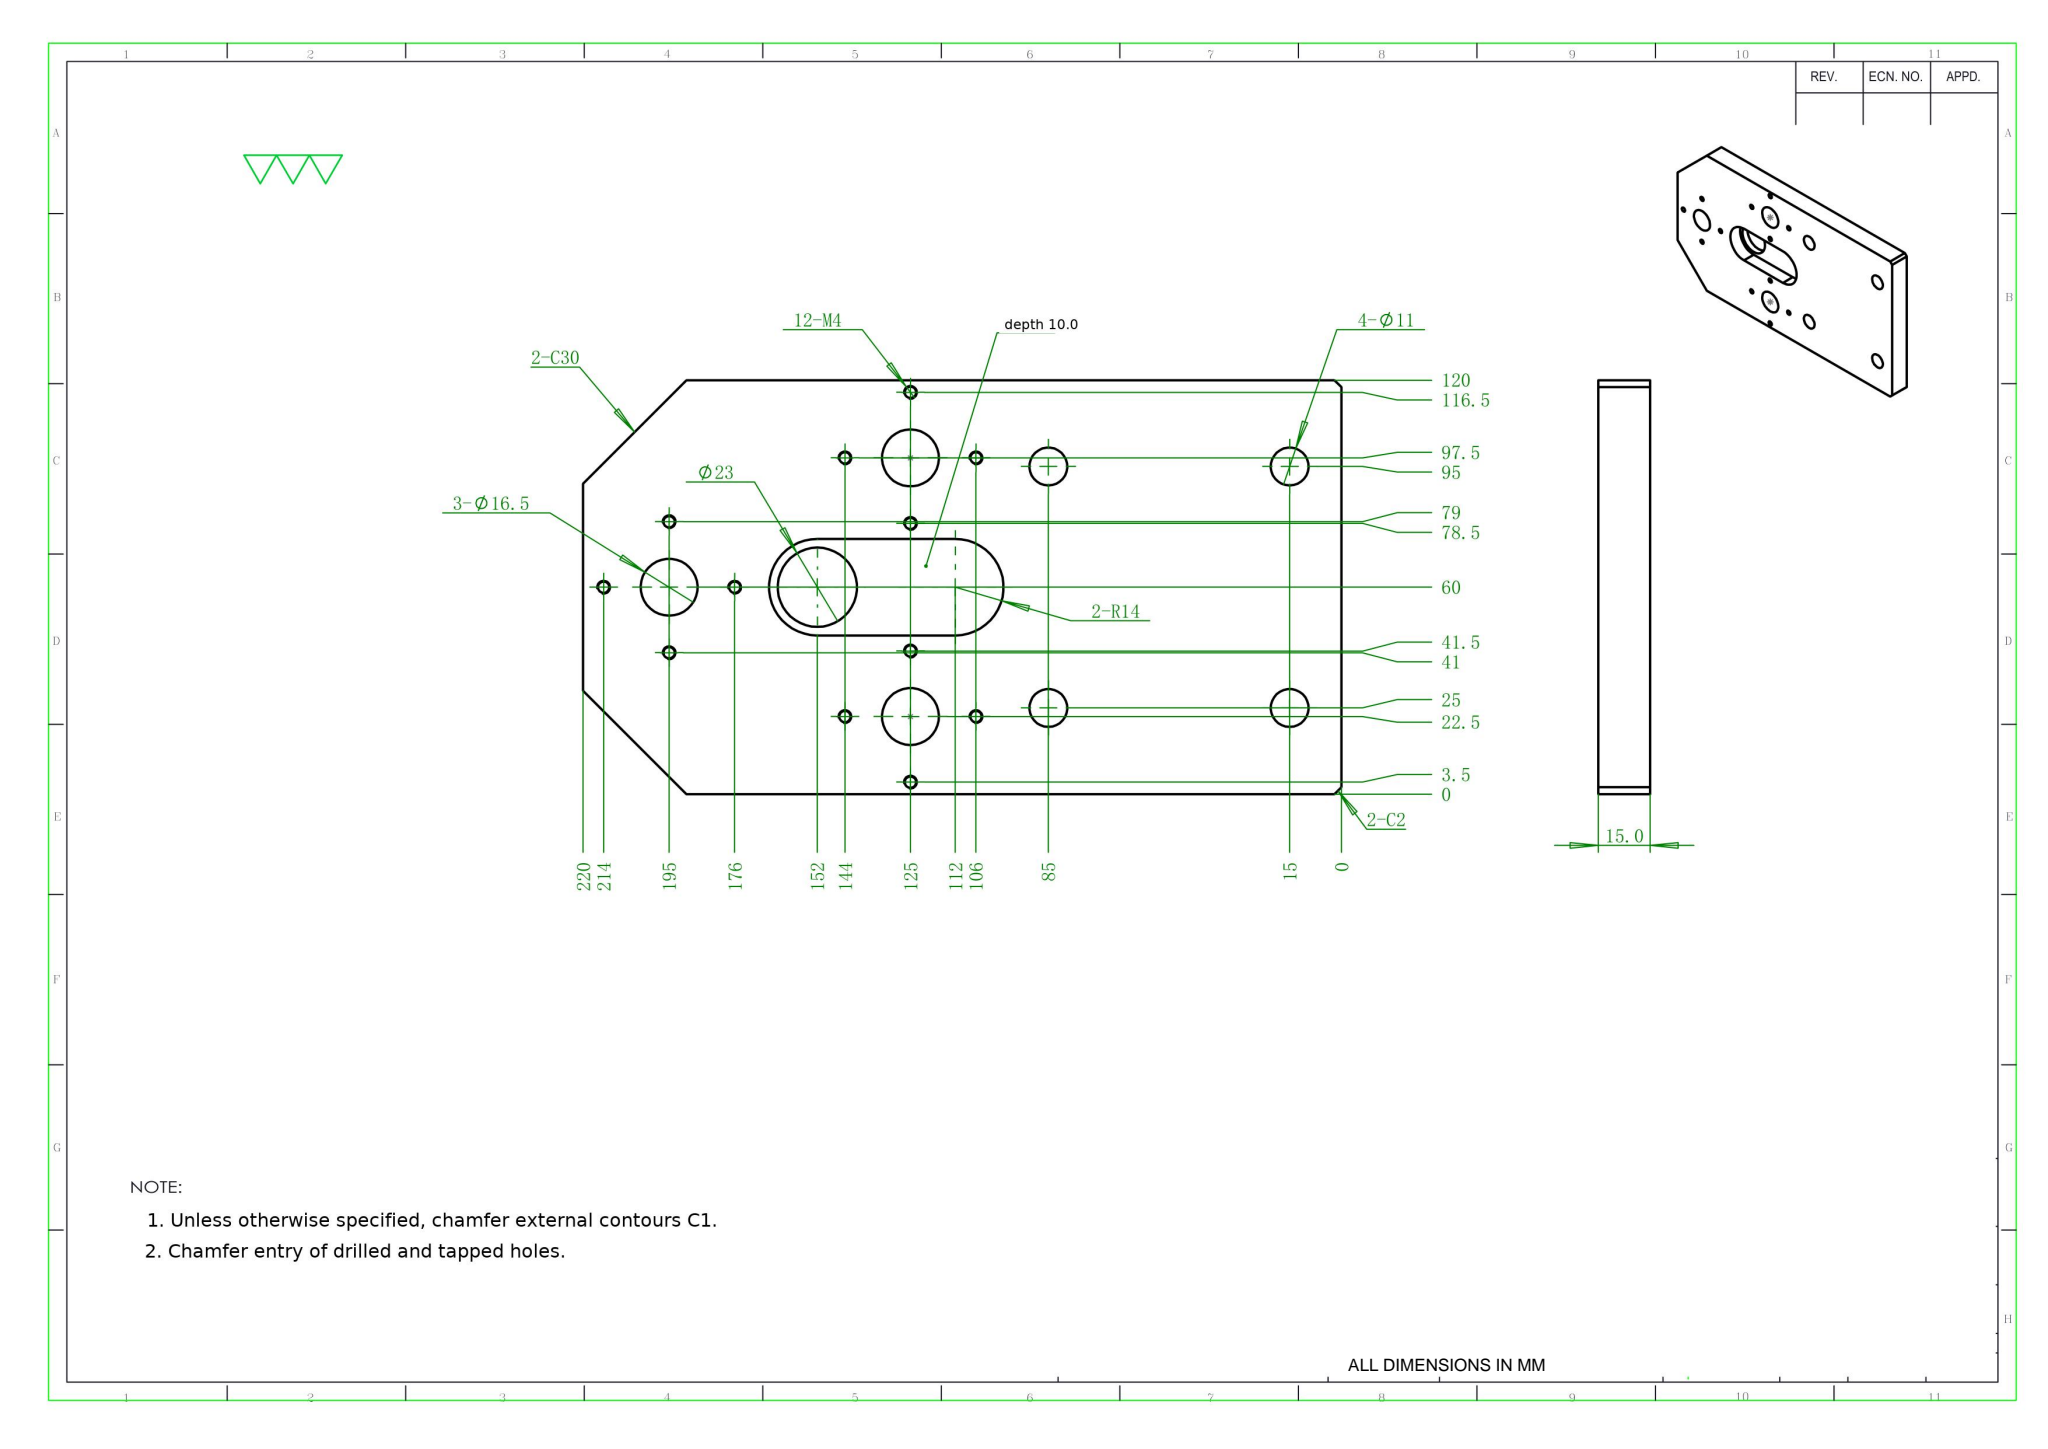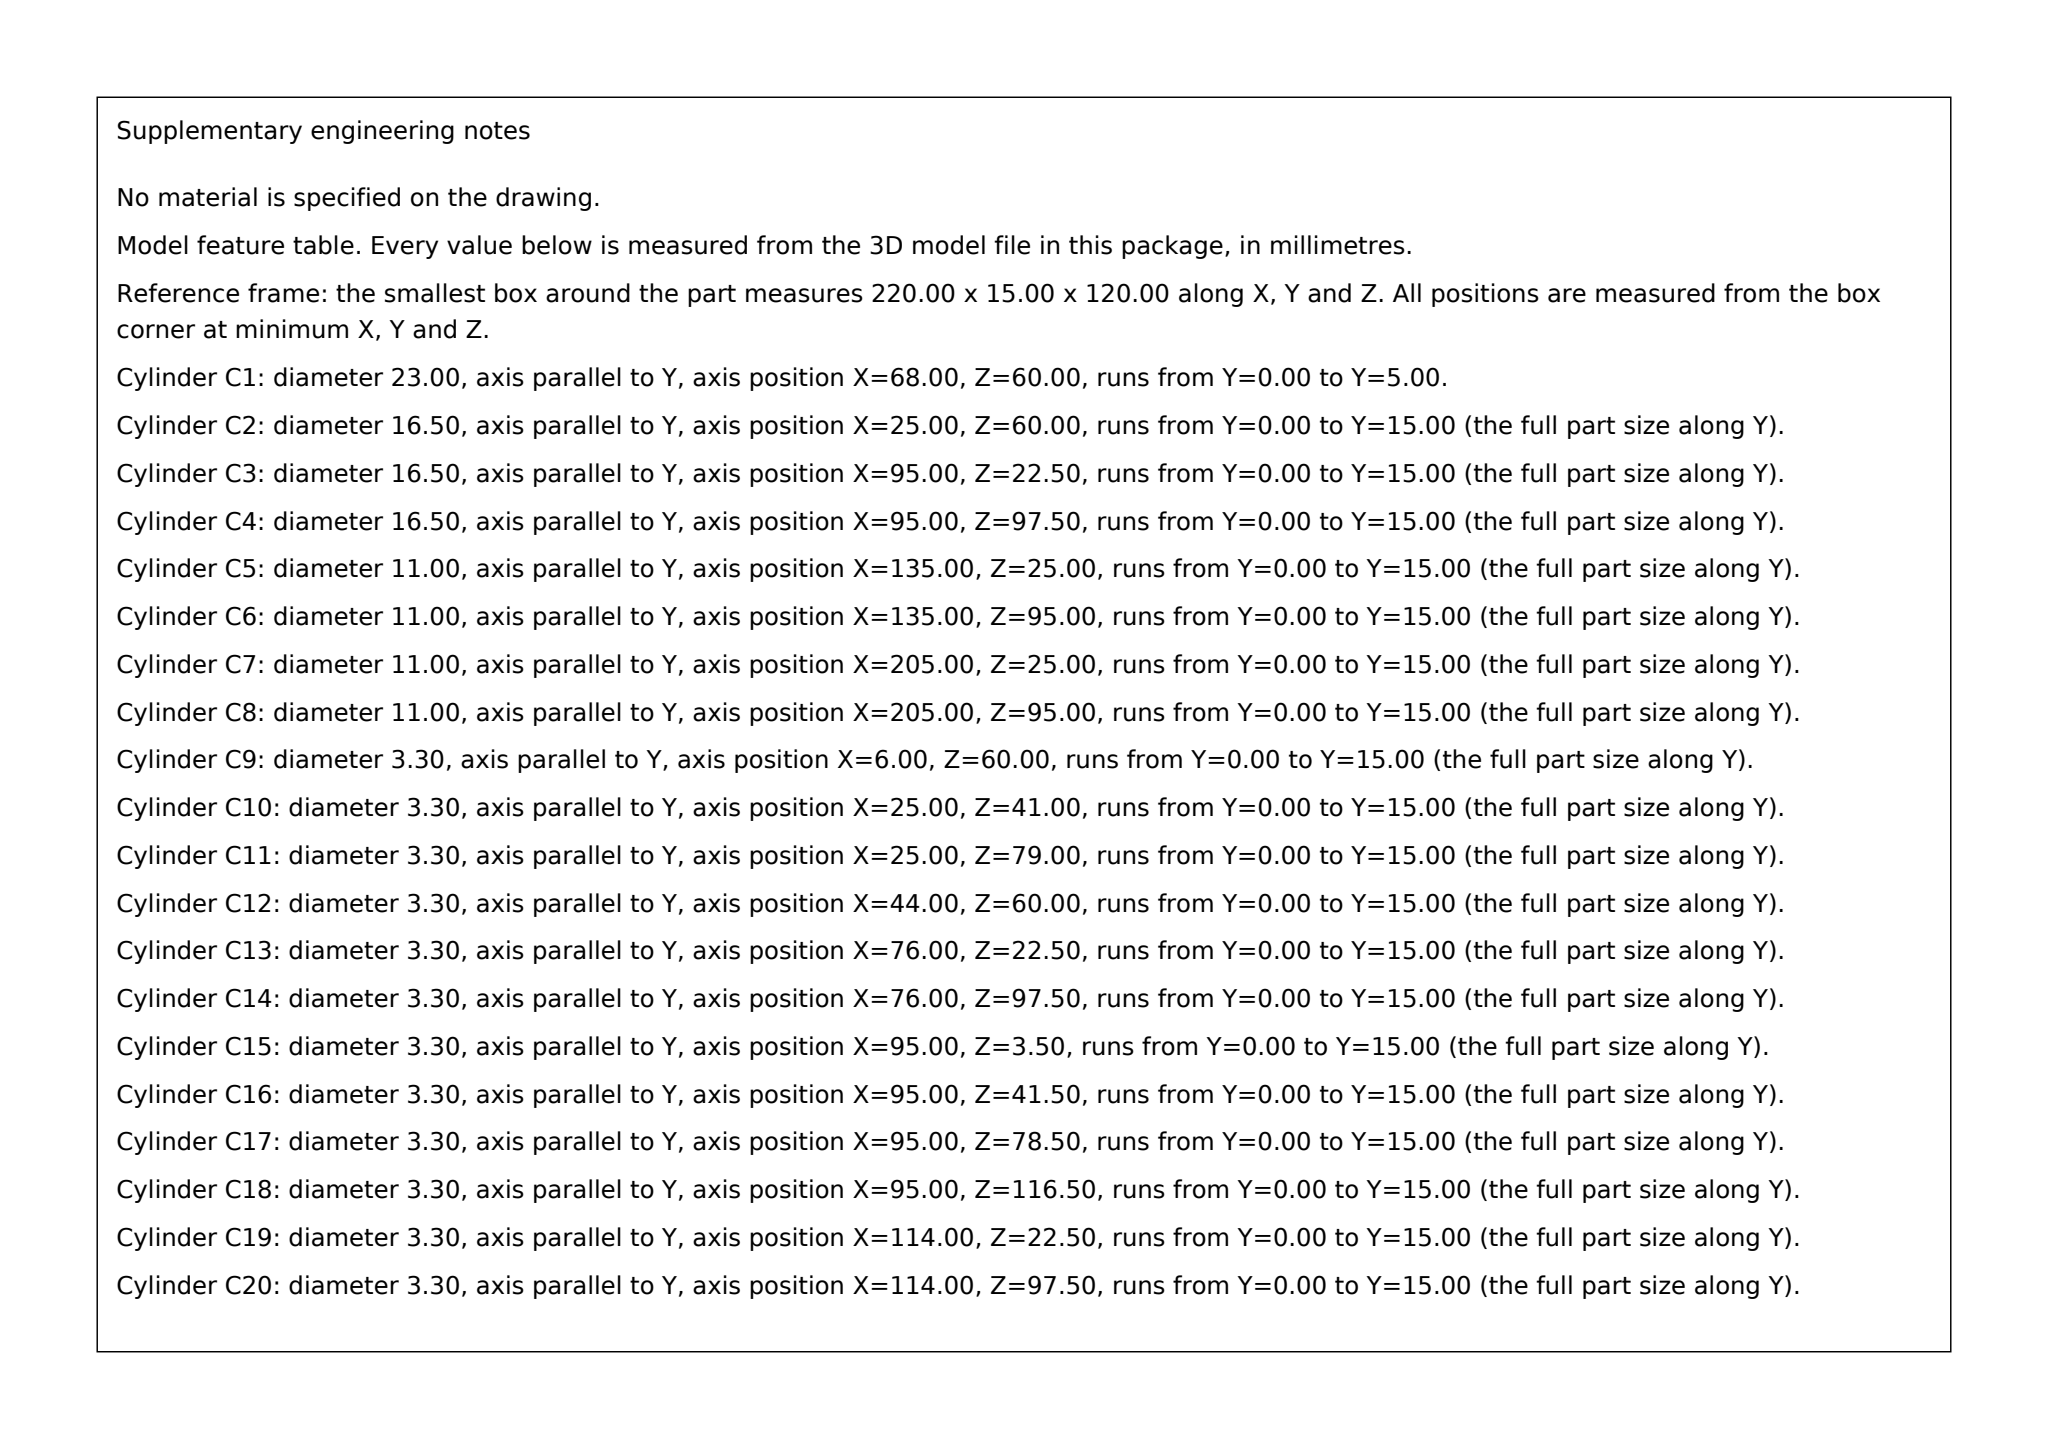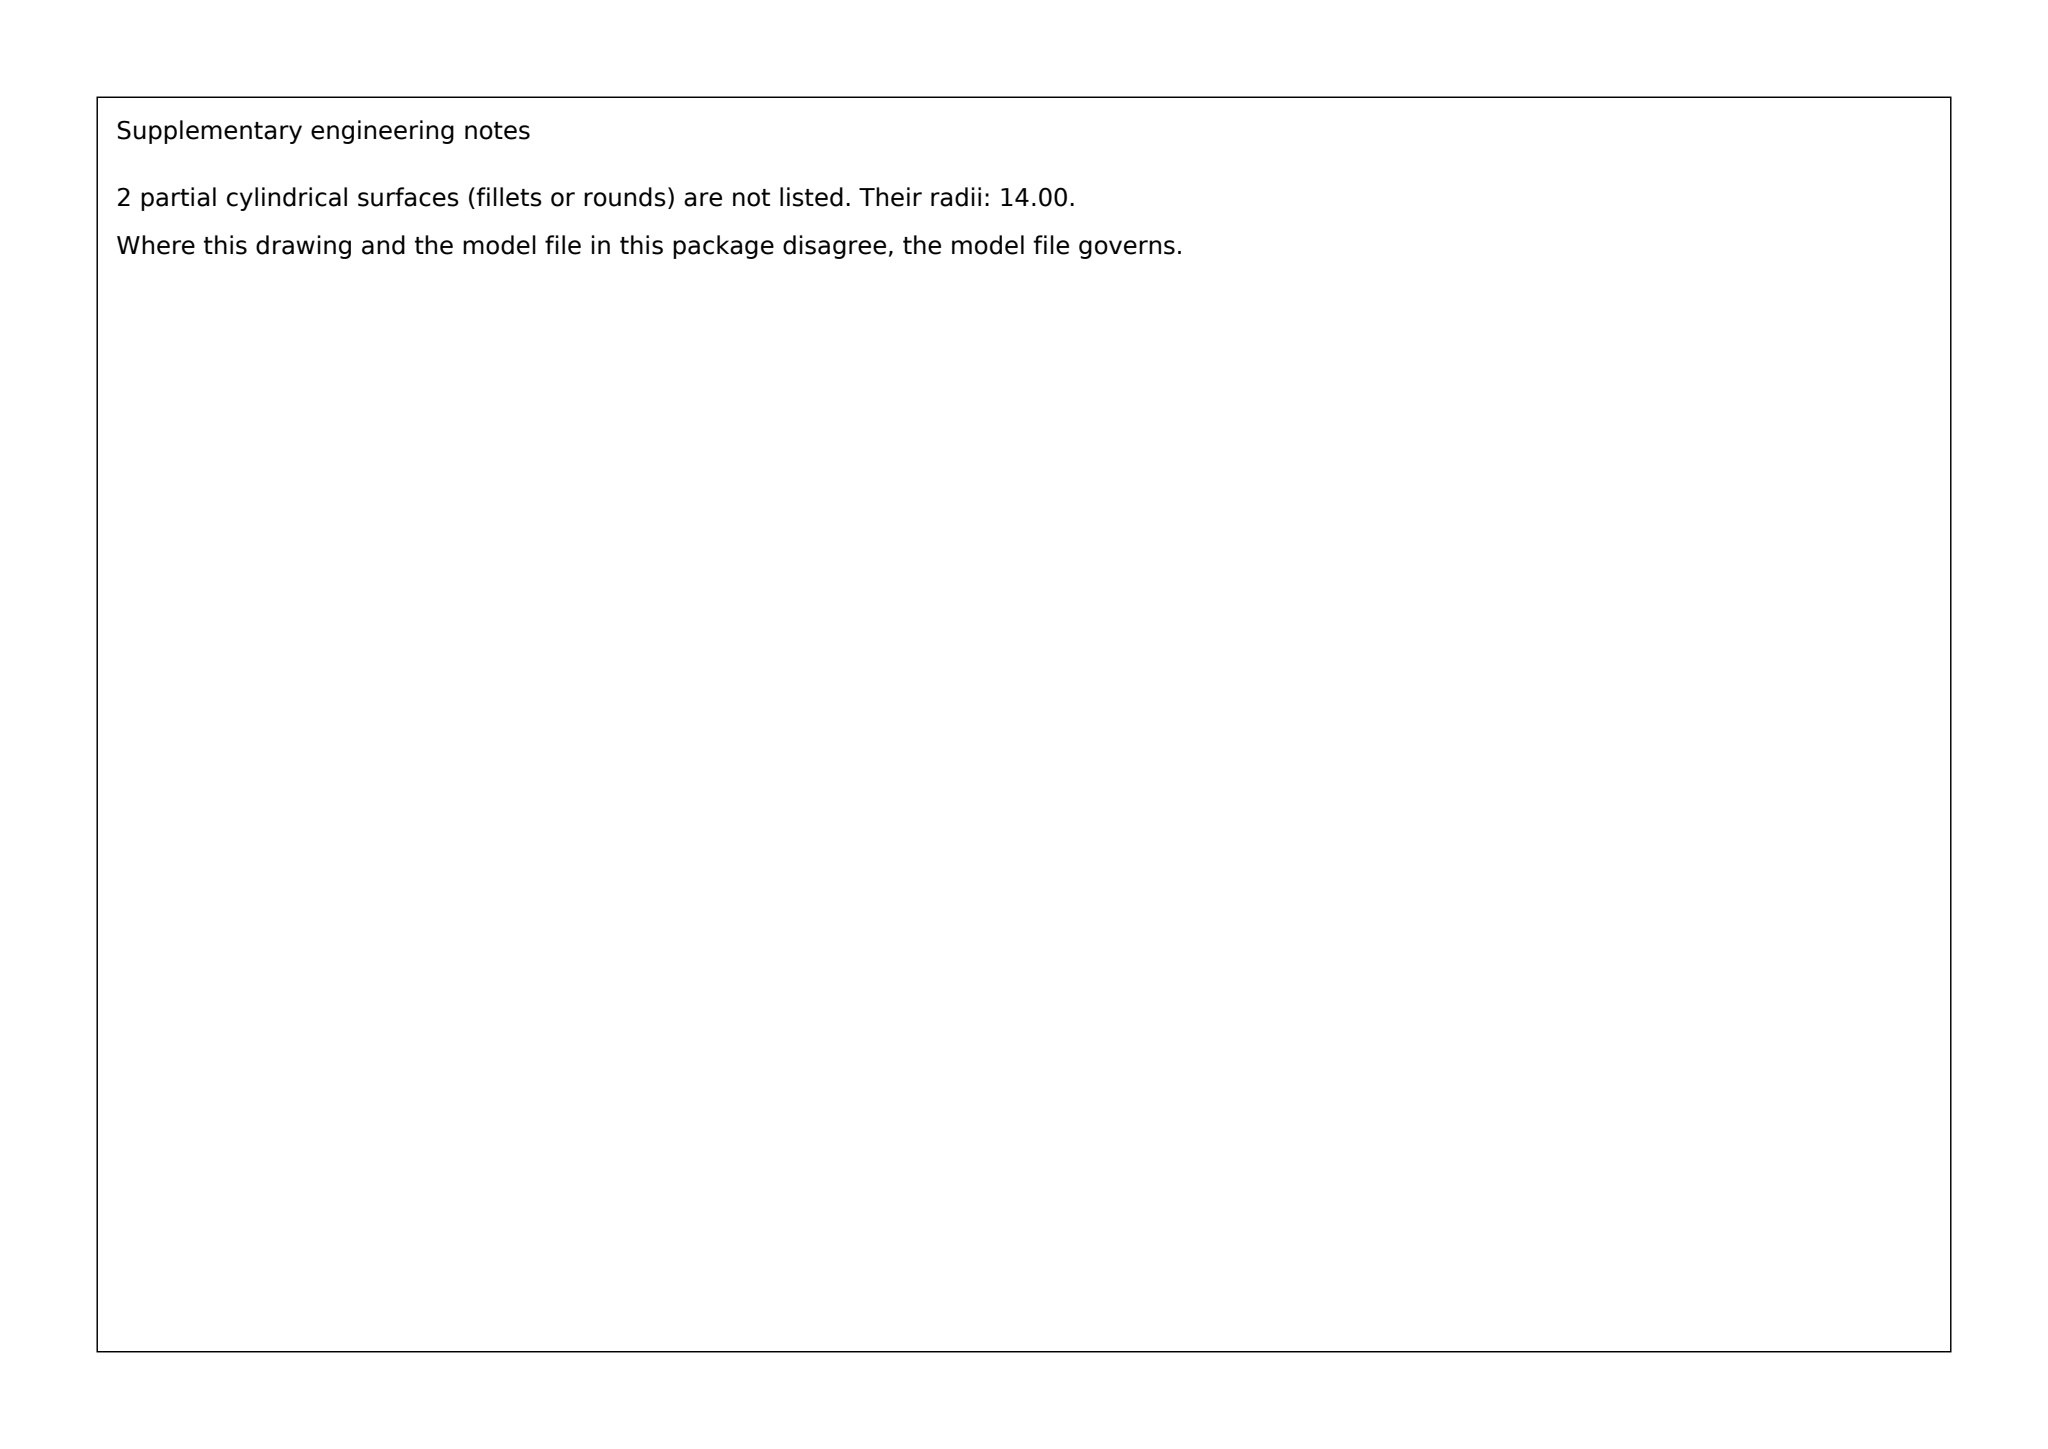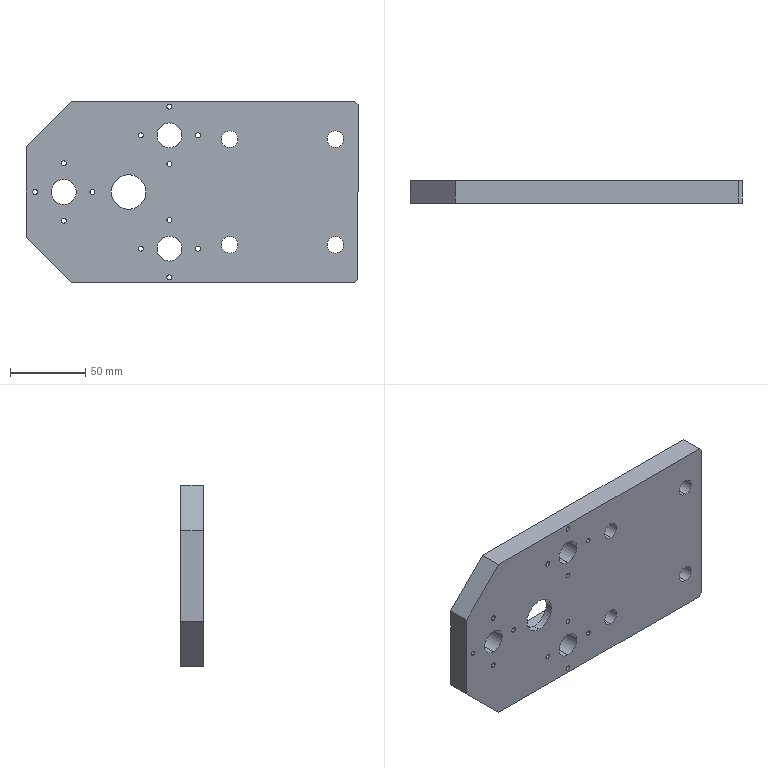Part | SolidWorks | mm | 1 solid | 55 faces | box 220 x 15 x 120 mm | volume 346141 mm3 | cylinder 42 | plane 13 | commonest cylinder face diameters 3.3 x24 11 x8 16.5 x6 23 x2 28 x2